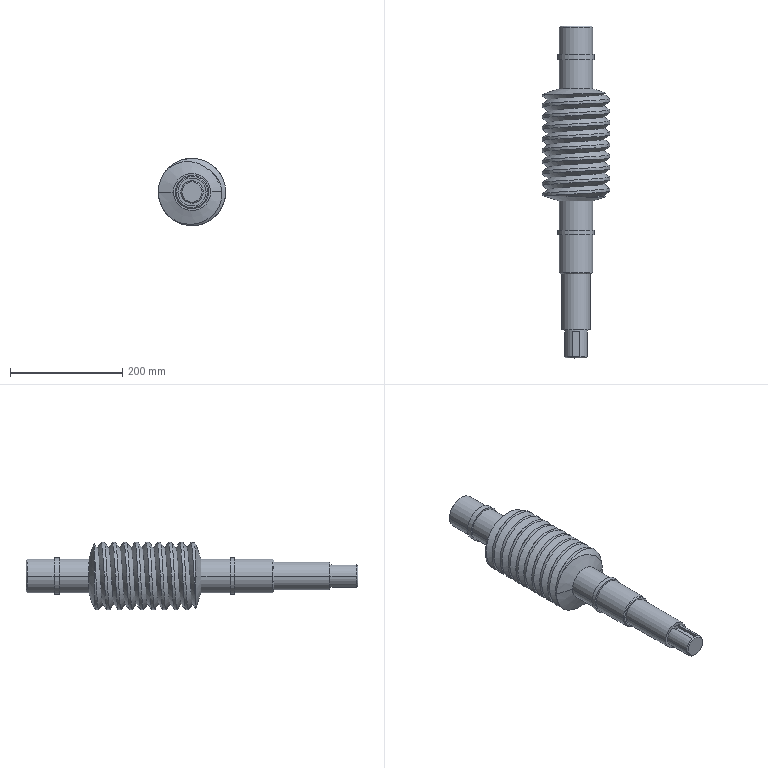Component | SolidWorks | WormShaft-1 | 1 solid | 61 faces | volume 2874619 mm3 | cylinder 36 | plane 13 | cone 10 | spline 2 | commonest cylinder face diameters 120 x20 60 x8 66 x4 40 x2 50 x2